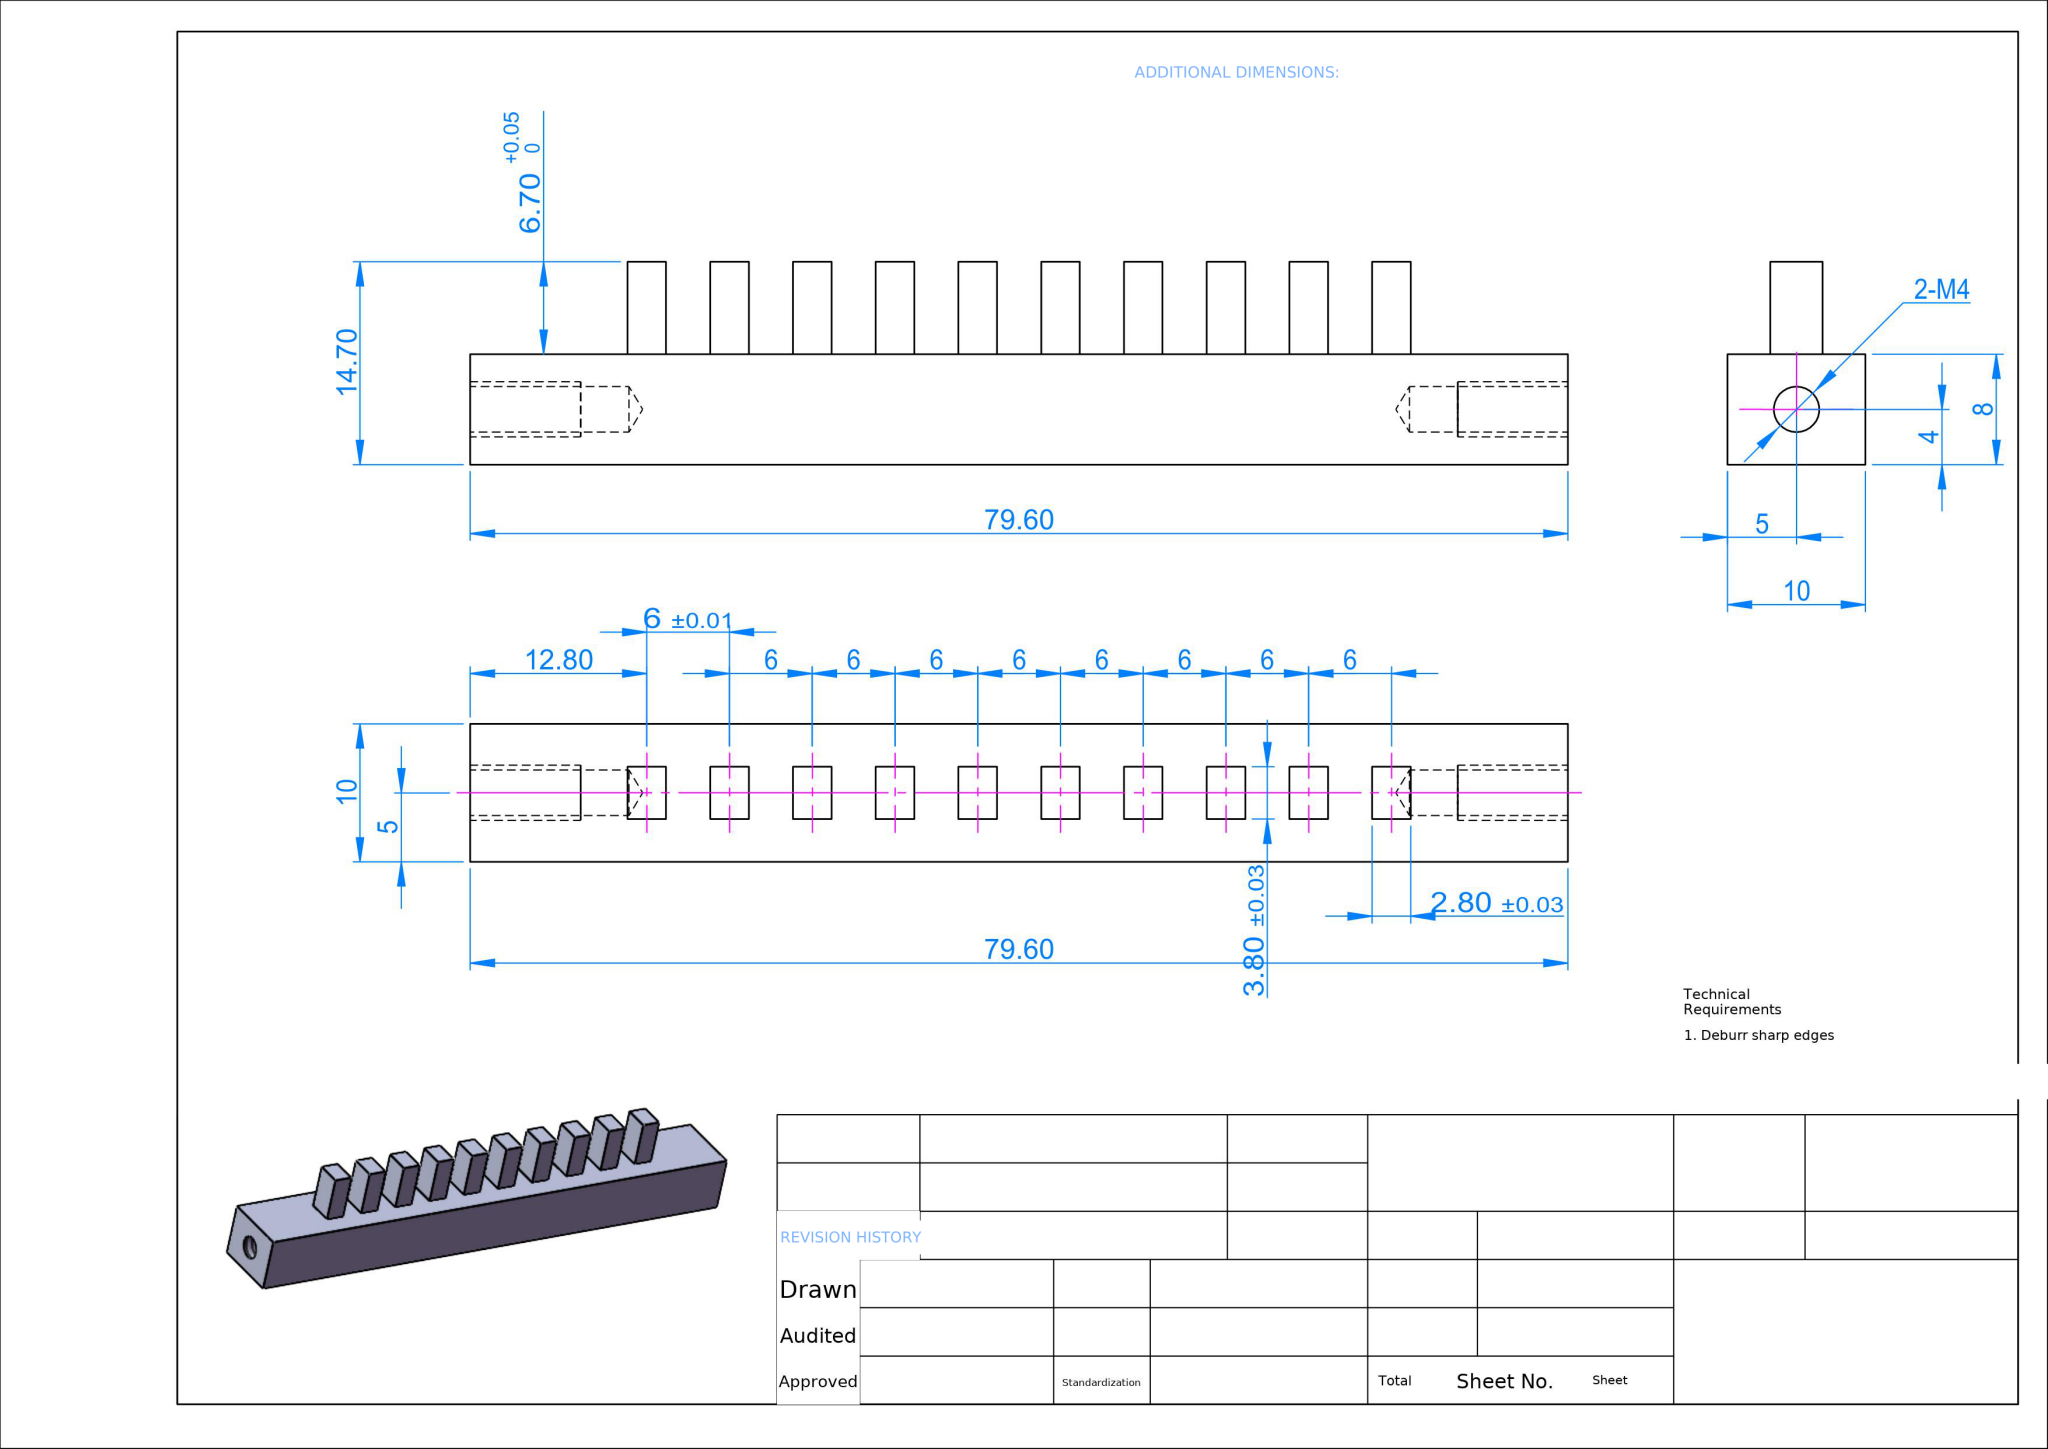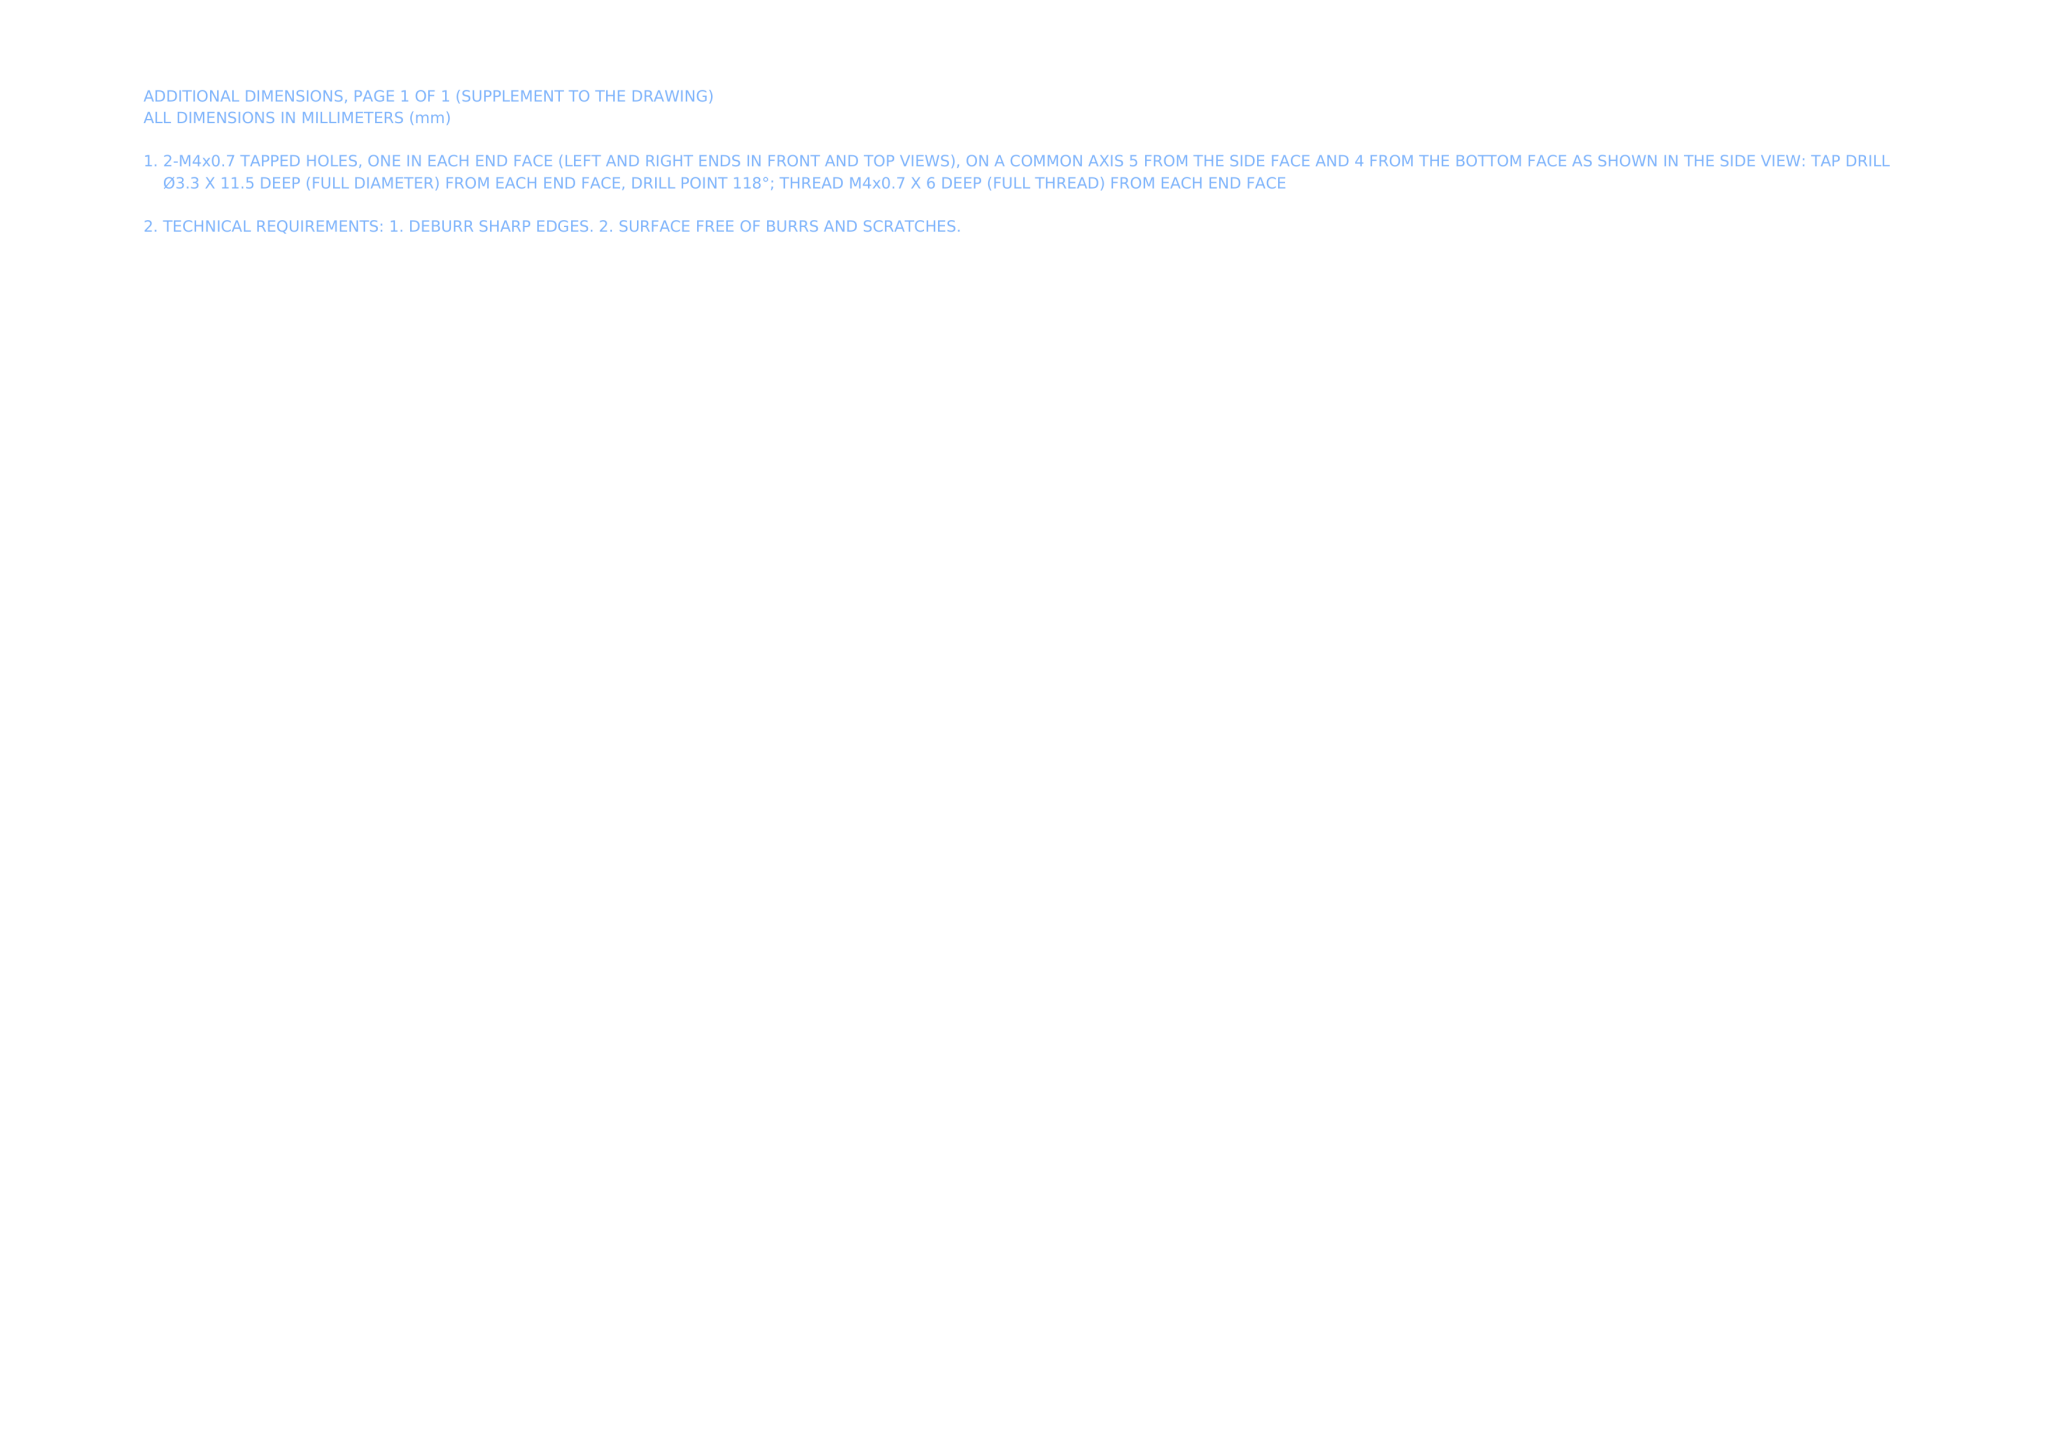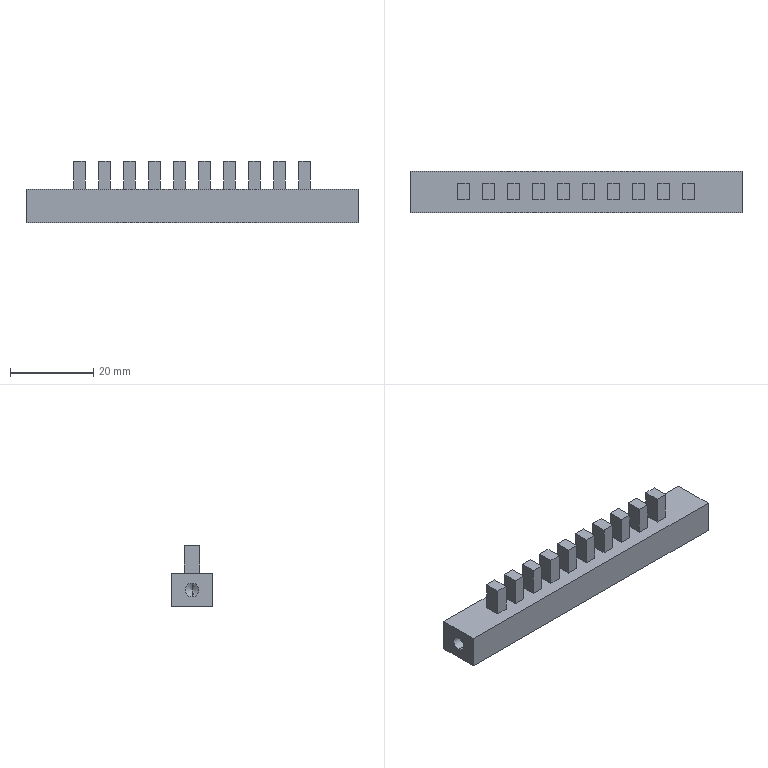Part | NX | mm | 1 solid | 64 faces | box 79.6 x 10 x 14.7 mm | volume 6879 mm3 | plane 56 | cylinder 4 | cone 4 | commonest cylinder face diameters 3.3 x4